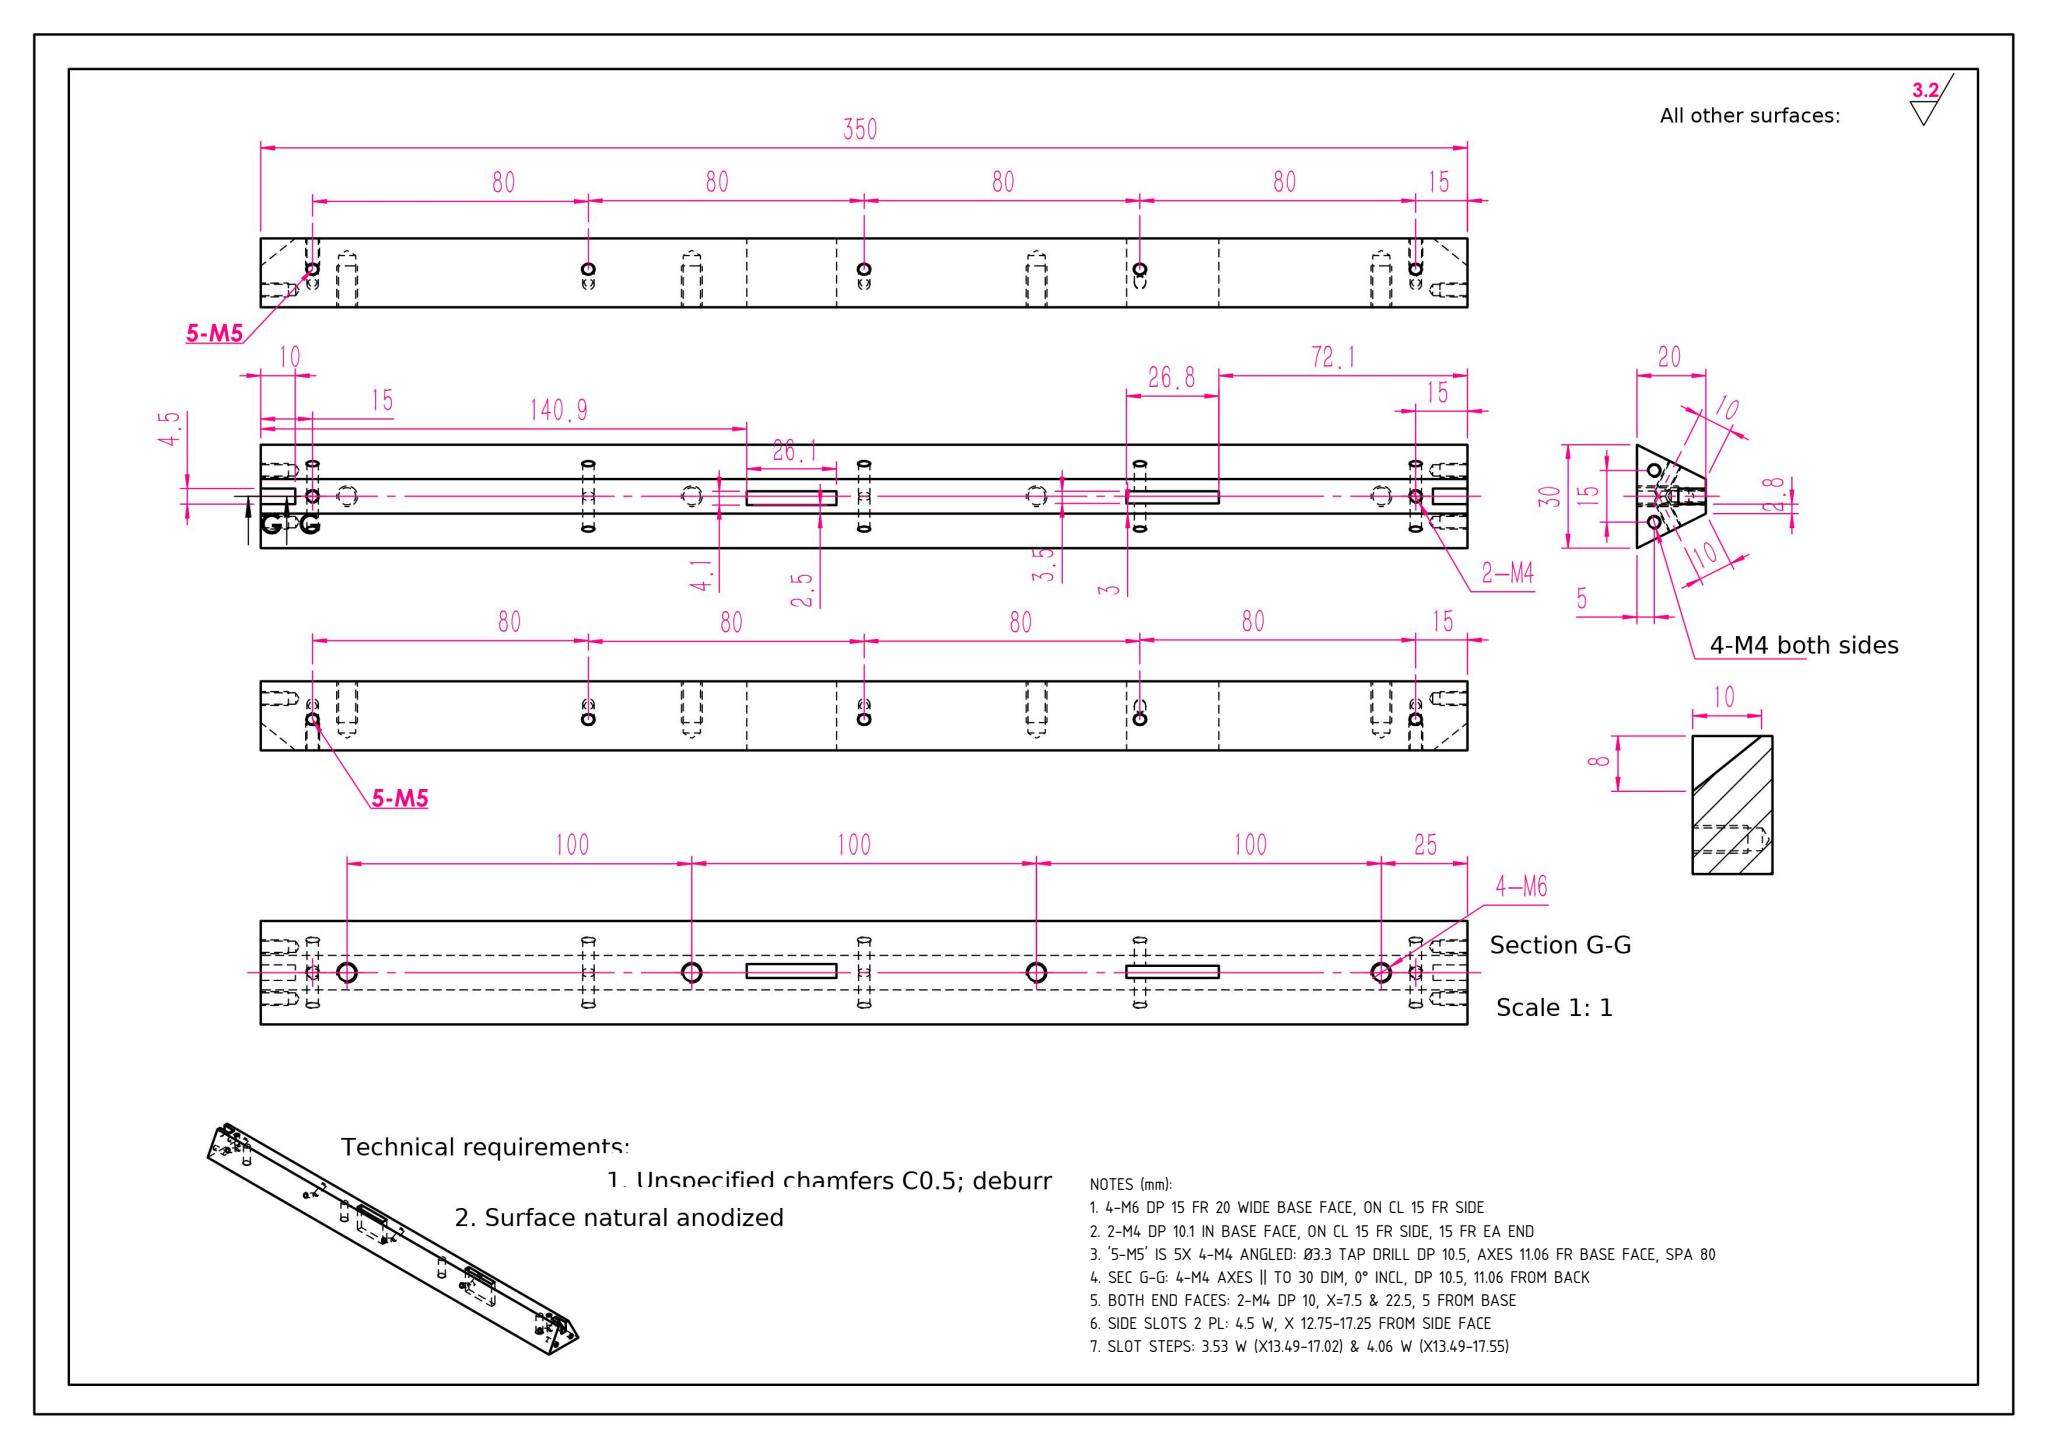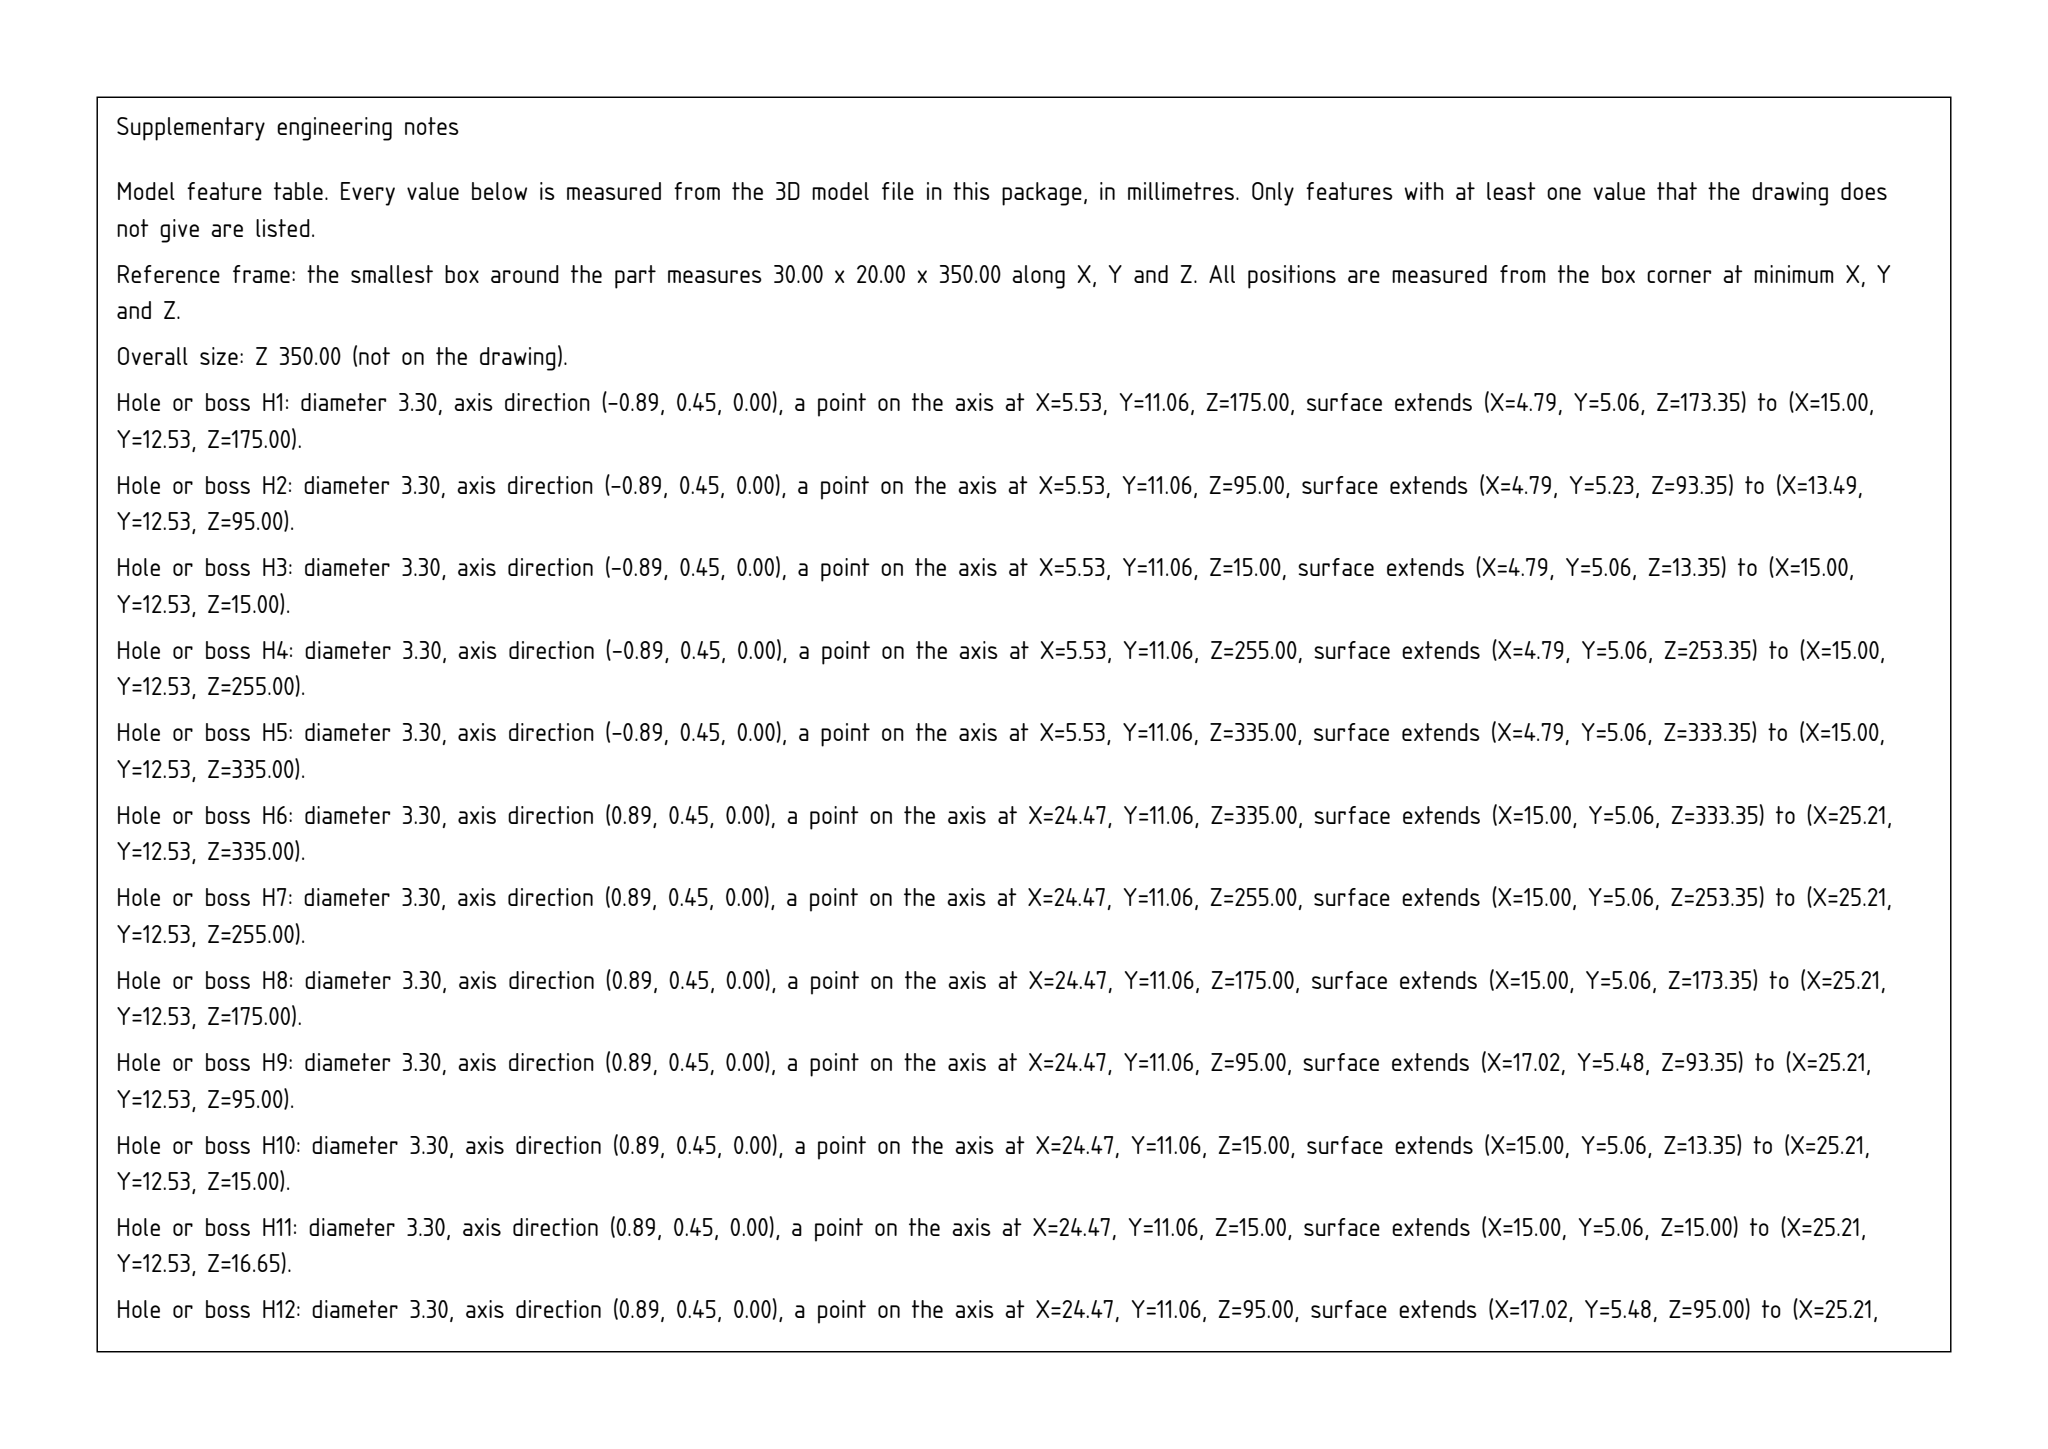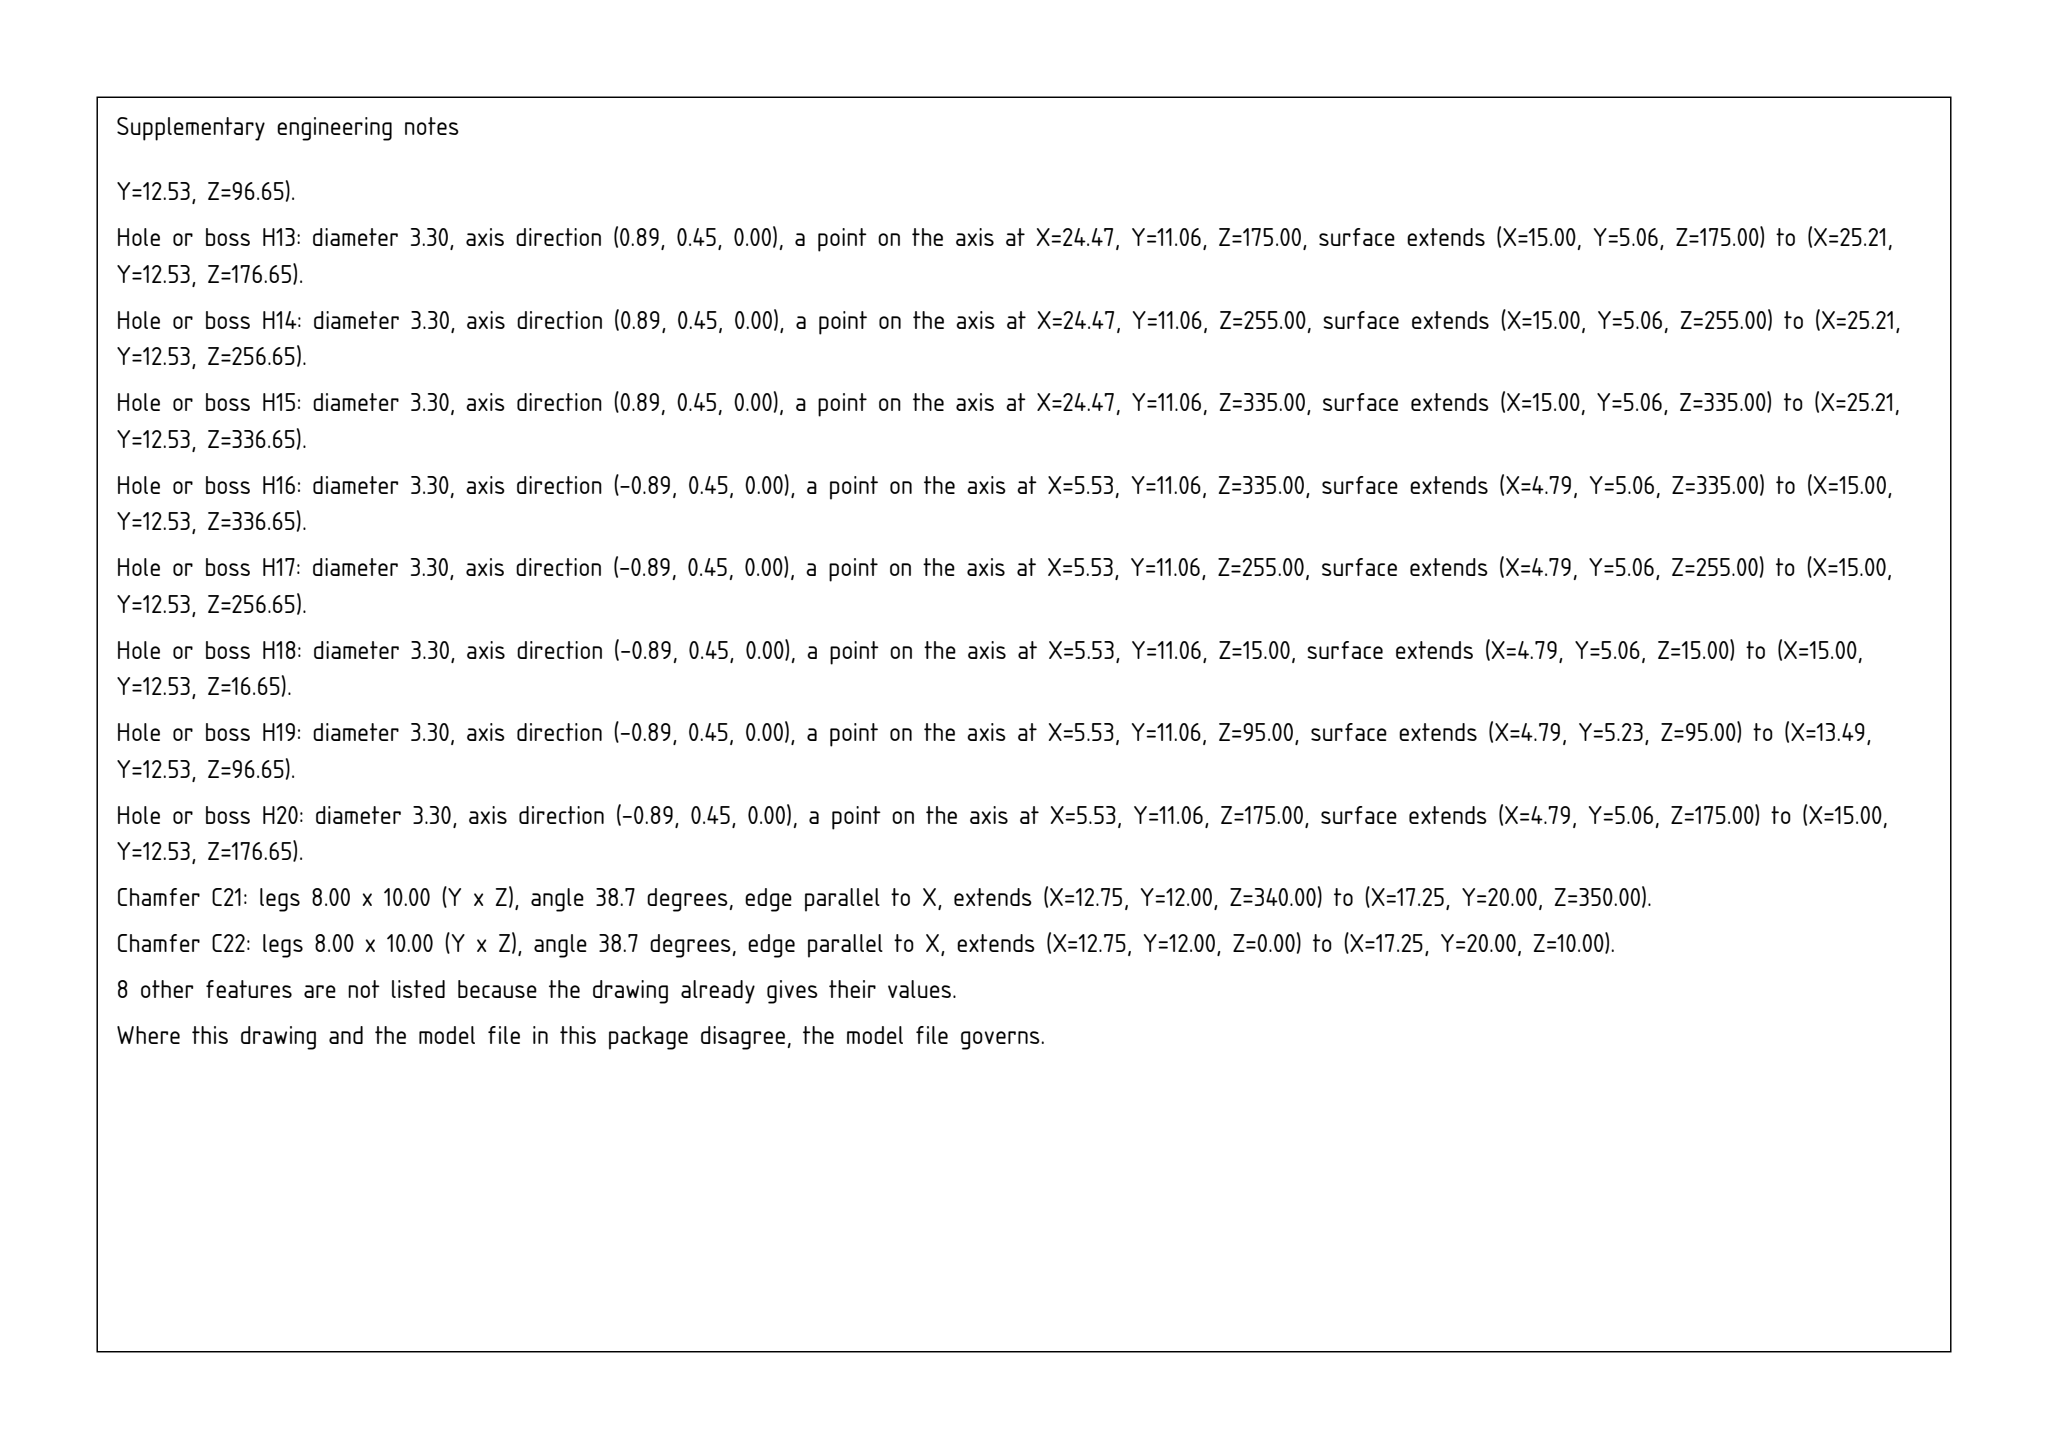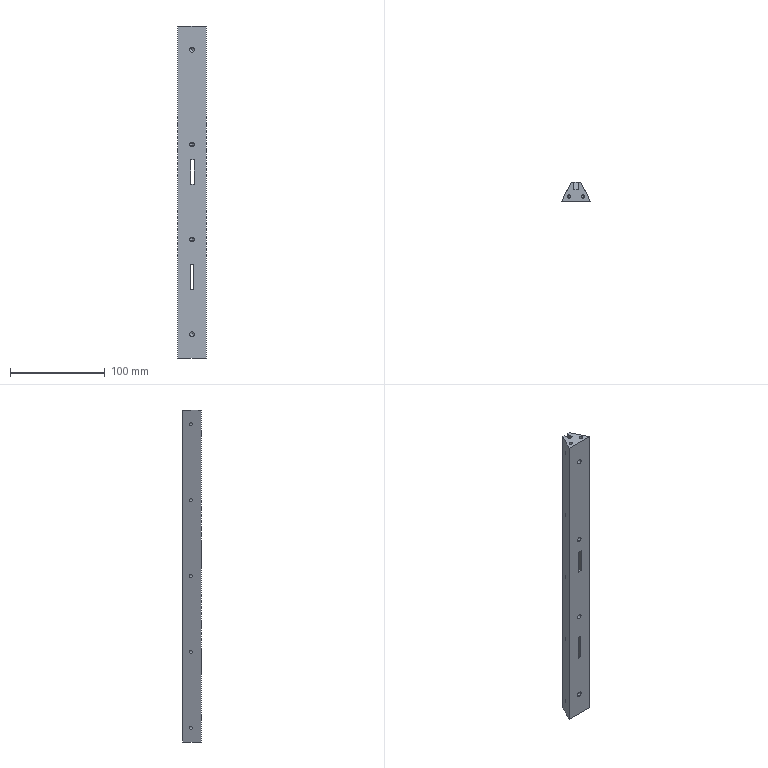Part | SolidWorks | mm | 1 solid | 92 faces | box 30 x 20 x 350 mm | volume 133032 mm3 | cylinder 40 | cone 32 | plane 20 | commonest cylinder face diameters 3.3 x32 5 x8
Drawing notes:
4-M6 DP 15 FR 20 WIDE BASE FACE, ON CL 15 FR SIDE | from the solid: Ø5.0 cyls, axis Y, x=15, z=25/125/225/325, length 15.0
2-M4 DP 10.1 IN BASE FACE, ON CL 15 FR SIDE, 15 FR EA END | from the solid: Ø3.3 cyls, axis Y, x=15, z=15 & 335, length 10.1
'5-M5' IS 5X 4-M4 ANGLED: Ø3.3 TAP DRILL DP 10.5, AXES 11.06 FR BASE FACE, SPA 80 | from the solid: Ø3.3 X-axis cyls len 10.51, y=11.06, z=15/95/175/255/335; no Ø4.2/M5 feature
SEC G-G: 4-M4 AXES || TO 30 DIM, 0° INCL, DP 10.5, 11.06 FROM BACK | from the solid: cylinders dia3.3 axis=x at y=11.06, z=15/95/175/255/335, len 10.51 (x-parallel, not inclined); 4 per station = 20 holes
BOTH END FACES: 2-M4 DP 10, X=7.5 & 22.5, 5 FROM BASE | from the solid: cylinders dia3.3 axis=z at [7.5,5.0] and [22.5,5.0], length 10.1; 118° drill cones ref dia 3.3
SIDE SLOTS 2 PL: 4.5 W, X 12.75-17.25 FROM SIDE FACE | from the solid: x-normal planes 12.75 (x2) and 17.25 (x2) => 4.50 width, sym about x=15 CL; slot lengths z 72.13-98.88 (26.75) and z 183.0-209.06 (26.06)
SLOT STEPS: 3.53 W (X13.49-17.02) & 4.06 W (X13.49-17.55) | from the solid: x-normal planes 13.49 (x2), 17.02 (x1), 17.55 (x1)
build123d program:
from build123d import *

# Parameters (mm, degrees)
BOSS_EXTRUDE1_DEPTH     = 350
M4_TAPPED_HOLE1_D       = 3.3
M4_TAPPED_HOLE1_DEPTH   = 10.1
M4_TAPPED_HOLE1_TIP     = 0.9914
M4_TAPPED_HOLE2_D       = 3.3
M4_TAPPED_HOLE2_DEPTH   = 10.1
M4_TAPPED_HOLE2_TIP     = 0.9914
M4_TAPPED_HOLE3_D       = 3.3
M4_TAPPED_HOLE3_DEPTH   = 10.1
M4_TAPPED_HOLE3_TIP     = 0.9914
M6_TAPPED_HOLE1_D       = 5
M6_TAPPED_HOLE1_DEPTH   = 15
M6_TAPPED_HOLE1_TIP     = 1.502
M4_TAPPED_HOLE4_D       = 3.3
M4_TAPPED_HOLE4_DEPTH   = 10.1
M4_TAPPED_HOLE4_TIP     = 0.9914
M4_TAPPED_HOLE5_D       = 3.3
M4_TAPPED_HOLE5_DEPTH   = 10.1
M4_TAPPED_HOLE5_TIP     = 0.9914
CUT_EXTRUDE1_DEPTH      = 2.25
CUT_EXTRUDE1_DEPTH_BACK = 2.25
SKETCH17_W              = 3.528
SKETCH17_H              = 26.751
SKETCH17_W_2            = 4.059
SKETCH17_H_2            = 26.06
CUT_EXTRUDE2_DEPTH      = 78


with BuildPart() as part:
    # Sketch1 → Boss-Extrude1 (new body)
    with BuildSketch(Plane.XY):
        Polygon((-5, 0), (5, 0), (15, -20), (-15, -20), align=None)
    extrude(amount=BOSS_EXTRUDE1_DEPTH)

    # M4 Tapped Hole1
    with Locations(Plane(origin=(4, 2, 0), x_dir=(0, 0, -1), z_dir=(0.8944, 0.4472, 0))):
        with Locations((-335, -12.236), (-255, -12.236), (-175, -12.236), (-95, -12.236), (-15, -12.236)):
            Hole(M4_TAPPED_HOLE1_D / 2, depth=M4_TAPPED_HOLE1_DEPTH)
            with Locations((0, 0, -(M4_TAPPED_HOLE1_DEPTH + M4_TAPPED_HOLE1_TIP / 2))):  # 118° drill point
                Cone(0, M4_TAPPED_HOLE1_D / 2, M4_TAPPED_HOLE1_TIP, mode=Mode.SUBTRACT)

    # M4 Tapped Hole2
    with Locations(Plane(origin=(-4, 2, 0), x_dir=(0, 0, 1), z_dir=(-0.8944, 0.4472, 0))):
        with Locations((175, -12.236), (95, -12.236), (15, -12.236), (255, -12.236), (335, -12.236)):
            Hole(M4_TAPPED_HOLE2_D / 2, depth=M4_TAPPED_HOLE2_DEPTH)
            with Locations((0, 0, -(M4_TAPPED_HOLE2_DEPTH + M4_TAPPED_HOLE2_TIP / 2))):  # 118° drill point
                Cone(0, M4_TAPPED_HOLE2_D / 2, M4_TAPPED_HOLE2_TIP, mode=Mode.SUBTRACT)

    # M4 Tapped Hole3
    with Locations(Plane(origin=(0, 0, 0), x_dir=(1, 0, 0), z_dir=(0, 1, 0))):
        with Locations((0, -15), (0, -335)):
            Hole(M4_TAPPED_HOLE3_D / 2, depth=M4_TAPPED_HOLE3_DEPTH)
            with Locations((0, 0, -(M4_TAPPED_HOLE3_DEPTH + M4_TAPPED_HOLE3_TIP / 2))):  # 118° drill point
                Cone(0, M4_TAPPED_HOLE3_D / 2, M4_TAPPED_HOLE3_TIP, mode=Mode.SUBTRACT)

    # M6 Tapped Hole1
    with Locations(Plane(origin=(0, -20, 0), x_dir=(-1, 0, 0), z_dir=(0, -1, 0))):
        with Locations((0, -325), (0, -225), (0, -125), (0, -25)):
            Hole(M6_TAPPED_HOLE1_D / 2, depth=M6_TAPPED_HOLE1_DEPTH)
            with Locations((0, 0, -(M6_TAPPED_HOLE1_DEPTH + M6_TAPPED_HOLE1_TIP / 2))):  # 118° drill point
                Cone(0, M6_TAPPED_HOLE1_D / 2, M6_TAPPED_HOLE1_TIP, mode=Mode.SUBTRACT)

    # M4 Tapped Hole4
    with Locations(Plane.XY.offset(350)):
        with Locations((-7.5, -15), (7.5, -15)):
            Hole(M4_TAPPED_HOLE4_D / 2, depth=M4_TAPPED_HOLE4_DEPTH)
            with Locations((0, 0, -(M4_TAPPED_HOLE4_DEPTH + M4_TAPPED_HOLE4_TIP / 2))):  # 118° drill point
                Cone(0, M4_TAPPED_HOLE4_D / 2, M4_TAPPED_HOLE4_TIP, mode=Mode.SUBTRACT)

    # M4 Tapped Hole5
    with Locations(Plane(origin=(0, 0, 0), x_dir=(-1, 0, 0), z_dir=(0, 0, -1))):
        with Locations((-7.5, -15), (7.5, -15)):
            Hole(M4_TAPPED_HOLE5_D / 2, depth=M4_TAPPED_HOLE5_DEPTH)
            with Locations((0, 0, -(M4_TAPPED_HOLE5_DEPTH + M4_TAPPED_HOLE5_TIP / 2))):  # 118° drill point
                Cone(0, M4_TAPPED_HOLE5_D / 2, M4_TAPPED_HOLE5_TIP, mode=Mode.SUBTRACT)

    # Sketch16 → Cut-Extrude1 (cut, two sides: drawn at the far end of the back side and taken through both)
    with BuildSketch(Plane(origin=(0, 0, 0), x_dir=(0, 0, -1), z_dir=(1, 0, 0)).offset(-CUT_EXTRUDE1_DEPTH_BACK)):
        Polygon((-350, -8), (-340, 0), (-350, 0), align=None)
        Polygon((0, -8), (-10, 0), (0, 0), align=None)
    extrude(amount=CUT_EXTRUDE1_DEPTH + CUT_EXTRUDE1_DEPTH_BACK, mode=Mode.SUBTRACT)

    # Sketch17 → Cut-Extrude2 (cut)
    with BuildSketch(Plane(origin=(0, 0, 0), x_dir=(1, 0, 0), z_dir=(0, 1, 0))):
        with Locations((0.252, -85.507)):
            Rectangle(SKETCH17_W, SKETCH17_H)
        with Locations((0.5171, -196.028)):
            Rectangle(SKETCH17_W_2, SKETCH17_H_2)
    extrude(amount=-CUT_EXTRUDE2_DEPTH, mode=Mode.SUBTRACT)


solid = part.part